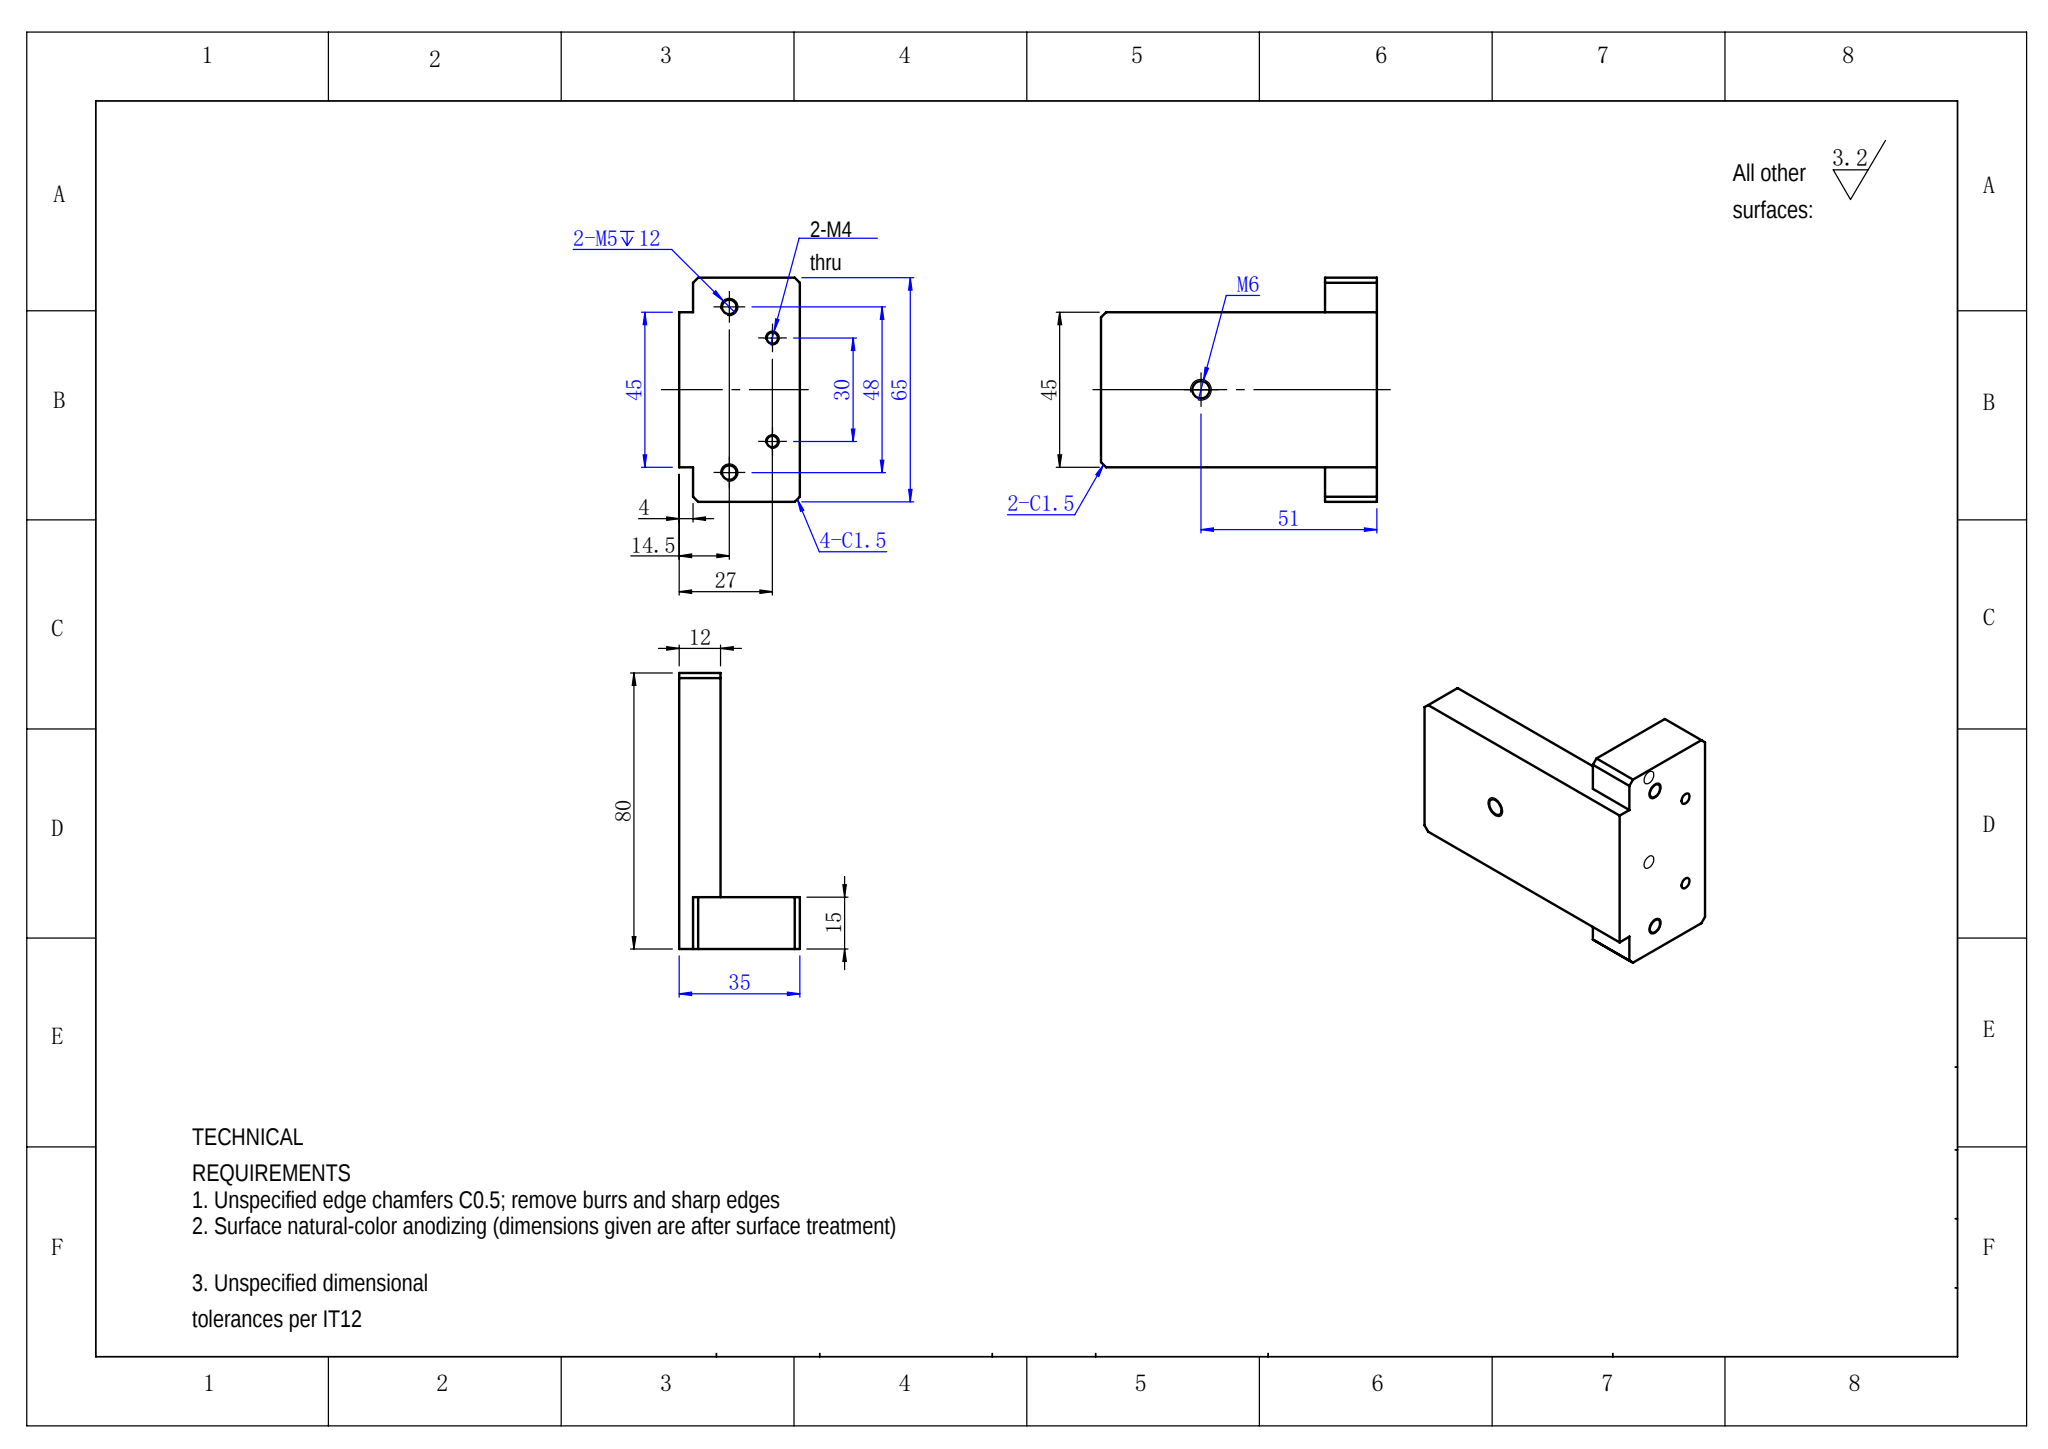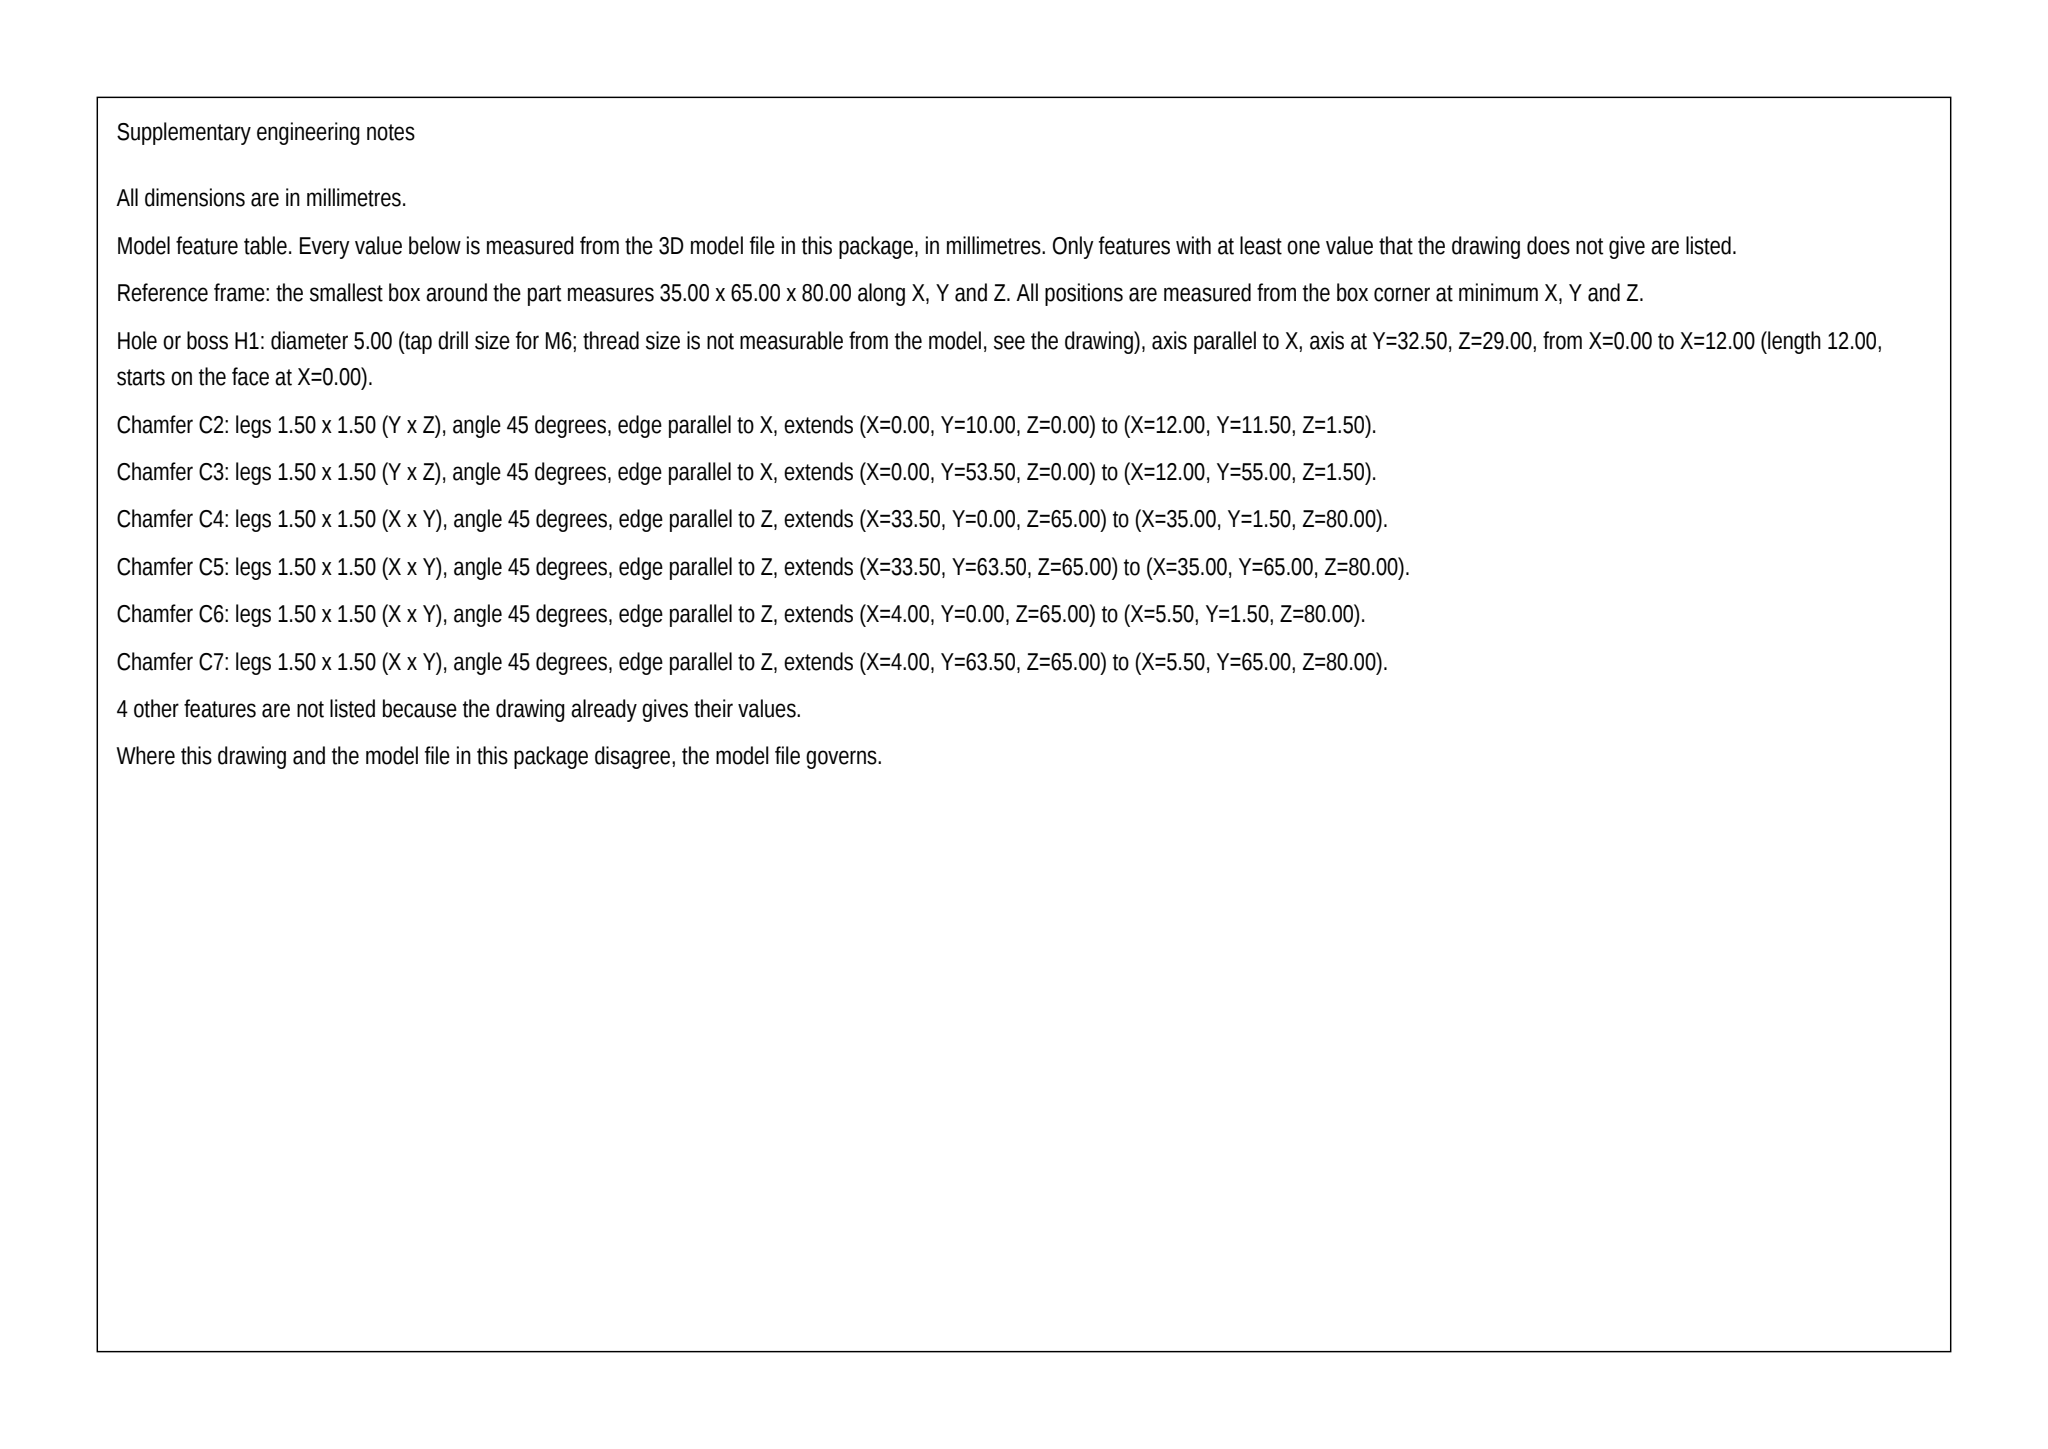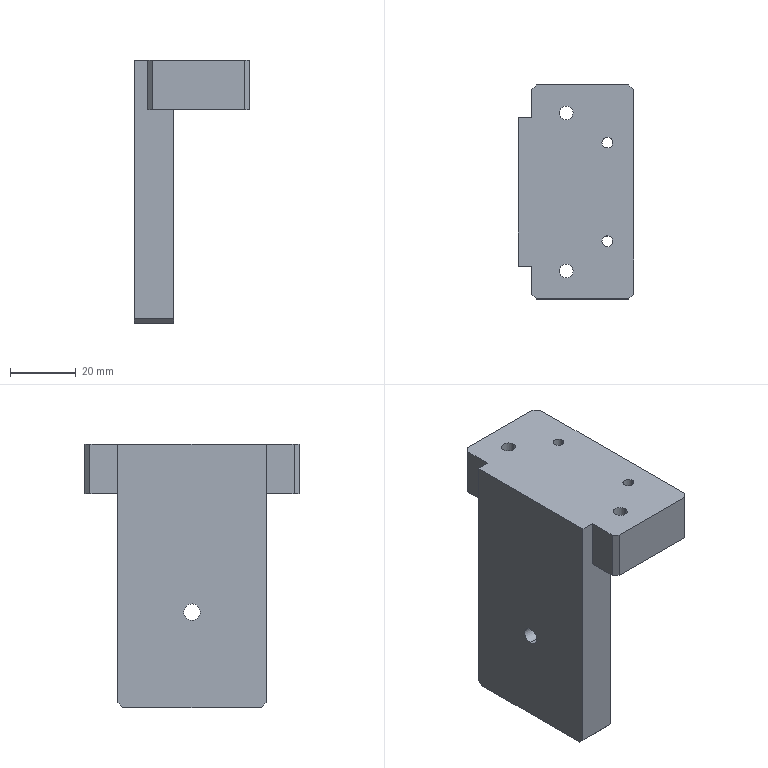Part | SolidWorks | mm | 1 solid | 28 faces | box 35 x 65 x 80 mm | volume 67023 mm3 | plane 18 | cylinder 10 | commonest cylinder face diameters 4.2 x4 3.3 x4 5 x2
build123d program:
from build123d import *

# Parameters (mm, degrees)
BOSS_EXTRUDE1_DEPTH   = 32.5
SKETCH13_W            = 4
SKETCH13_H            = 10
CUT_EXTRUDE5_DEPTH    = 94.173
SKETCH14_W            = 65
SKETCH14_H            = 10
CUT_EXTRUDE6_DEPTH    = 94.173
M6_TAPPED_HOLE1_D     = 5
M4_TAPPED_HOLE1_D     = 3.3
M5_TAPPED_HOLE1_D     = 4.2
M5_TAPPED_HOLE1_DEPTH = 16
M5_TAPPED_HOLE1_TIP   = 1.262
CHAMFER1_SIZE         = 1.5


with BuildPart() as part:
    # Sketch1 → Boss-Extrude1 (new, symmetric)
    with BuildSketch(Plane(origin=(0, 0, 0), x_dir=(1, 0, 0), z_dir=(0, 1, 0))):
        Polygon((0, 80), (0, 0), (35, 0), (35, 15), (12, 15), (12, 80), align=None)
    extrude(amount=BOSS_EXTRUDE1_DEPTH, both=True)

    # Sketch13 → Cut-Extrude5 (cut, through all)
    with BuildSketch(Plane.XY):
        with Locations((2, 27.5)):
            Rectangle(SKETCH13_W, SKETCH13_H)
        with Locations((2, -27.5)):
            Rectangle(SKETCH13_W, SKETCH13_H)
    extrude(amount=-CUT_EXTRUDE5_DEPTH, mode=Mode.SUBTRACT)

    # Sketch14 → Cut-Extrude6 (cut, through all)
    with BuildSketch(Plane.ZY):
        with Locations((-47.5, 27.5)):
            Rectangle(SKETCH14_W, SKETCH14_H)
        with Locations((-47.5, -27.5)):
            Rectangle(SKETCH14_W, SKETCH14_H)
    extrude(amount=-CUT_EXTRUDE6_DEPTH, mode=Mode.SUBTRACT)

    # M6 Tapped Hole1 (through all)
    with Locations(Plane.ZY):
        with Locations((-51, 0)):
            Hole(M6_TAPPED_HOLE1_D / 2)

    # M4 Tapped Hole1 (through all)
    with Locations(Plane(origin=(0, 0, -15), x_dir=(-1, 0, 0), z_dir=(0, 0, -1))):
        with Locations((-27, -15), (-27, 15)):
            Hole(M4_TAPPED_HOLE1_D / 2)

    # M5 Tapped Hole1
    with Locations(Plane.XY):
        with Locations((14.5, 24), (14.5, -24)):
            Hole(M5_TAPPED_HOLE1_D / 2, depth=M5_TAPPED_HOLE1_DEPTH)
            with Locations((0, 0, -(M5_TAPPED_HOLE1_DEPTH + M5_TAPPED_HOLE1_TIP / 2))):  # 118° drill point
                Cone(0, M5_TAPPED_HOLE1_D / 2, M5_TAPPED_HOLE1_TIP, mode=Mode.SUBTRACT)

    # Chamfer1
    chamfer1_edges = [part.edges().sort_by_distance(p)[0] for p in [
        (35, 32.5, -7.5),
        (6, 22.5, -80),
        (6, -22.5, -80),
        (4, 32.5, -7.5),
        (4, -32.5, -7.5),
        (35, -32.5, -7.5),
    ]]
    chamfer(chamfer1_edges, length=CHAMFER1_SIZE)


solid = part.part